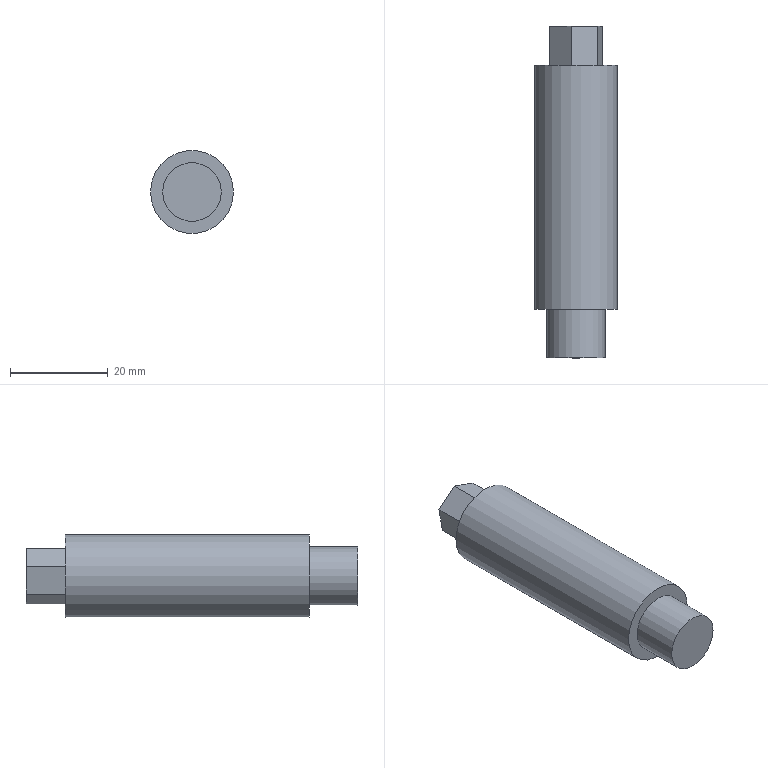Component | NX | STOP_PIN | 1 solid | 12 faces | box 17 x 68 x 17 mm | volume 13173 mm3 | plane 10 | cylinder 2 | commonest cylinder face diameters 12 x1 17 x1
STEP:
#1=CARTESIAN_POINT('',(0.,0.,0.));
#2=DIRECTION('',(0.,0.,1.));
#3=DIRECTION('',(1.,0.,0.));
#4=AXIS2_PLACEMENT_3D('',#1,#2,#3);
#5=CARTESIAN_POINT('',(-15.459,67.5,12.621));
#6=VERTEX_POINT('',#5);
#7=CARTESIAN_POINT('',(-6.959,67.5,12.621));
#8=DIRECTION('',(0.,-1.,0.));
#9=DIRECTION('',(-1.,0.,0.));
#10=AXIS2_PLACEMENT_3D('',#7,#8,#9);
#11=CIRCLE('',#10,8.5);
#12=CARTESIAN_POINT('',(-6.959,67.5,12.621));
#13=DIRECTION('',(0.,-1.,0.));
#14=DIRECTION('',(-1.,0.,0.));
#15=AXIS2_PLACEMENT_3D('',#12,#13,#14);
#16=PLANE('',#15);
#17=CARTESIAN_POINT('',(0.,0.));
#18=DIRECTION('',(1.,0.));
#19=AXIS2_PLACEMENT_2D('',#17,#18);
#20=CIRCLE('',#19,8.5);
#21=(GEOMETRIC_REPRESENTATION_CONTEXT(2)PARAMETRIC_REPRESENTATION_CONTEXT()REPRESENTATION_CONTEXT('',''));
#22=DEFINITIONAL_REPRESENTATION('',(#20),#21);
#23=PCURVE('',#16,#22);
#24=CARTESIAN_POINT('',(-6.959,67.5,12.621));
#25=DIRECTION('',(0.,-1.,0.));
#26=DIRECTION('',(-1.,0.,0.));
#27=AXIS2_PLACEMENT_3D('',#24,#25,#26);
#28=CYLINDRICAL_SURFACE('',#27,8.5);
#29=CARTESIAN_POINT('',(0.,0.));
#30=DIRECTION('',(1.,0.));
#31=VECTOR('',#30,1.);
#32=LINE('',#29,#31);
#33=(GEOMETRIC_REPRESENTATION_CONTEXT(2)PARAMETRIC_REPRESENTATION_CONTEXT()REPRESENTATION_CONTEXT('',''));
#34=DEFINITIONAL_REPRESENTATION('',(#32),#33);
#35=PCURVE('',#28,#34);
#36=SURFACE_CURVE('',#11,(#23,#35),.PCURVE_S1.);
#37=EDGE_CURVE('',#6,#6,#36,.T.);
#38=ORIENTED_EDGE('',*,*,#37,.F.);
#39=EDGE_LOOP('',(#38));
#40=FACE_BOUND('',#39,.T.);
#41=CARTESIAN_POINT('',(-7.962,67.5,18.307));
#42=VERTEX_POINT('',#41);
#43=CARTESIAN_POINT('',(-2.537,67.5,16.333));
#44=VERTEX_POINT('',#43);
#45=CARTESIAN_POINT('',(-7.962,67.5,18.307));
#46=DIRECTION('',(0.9397,0.,-0.342));
#47=VECTOR('',#46,1.);
#48=LINE('',#45,#47);
#49=CARTESIAN_POINT('',(1.003,-5.686));
#50=DIRECTION('',(-0.9397,0.342));
#51=VECTOR('',#50,1.);
#52=LINE('',#49,#51);
#53=(GEOMETRIC_REPRESENTATION_CONTEXT(2)PARAMETRIC_REPRESENTATION_CONTEXT()REPRESENTATION_CONTEXT('',''));
#54=DEFINITIONAL_REPRESENTATION('',(#52),#53);
#55=PCURVE('',#16,#54);
#56=CARTESIAN_POINT('',(-7.962,75.5,18.307));
#57=DIRECTION('',(-0.342,0.,-0.9397));
#58=DIRECTION('',(-0.9397,0.,0.342));
#59=AXIS2_PLACEMENT_3D('',#56,#57,#58);
#60=PLANE('',#59);
#61=CARTESIAN_POINT('',(0.,-8.));
#62=DIRECTION('',(-1.,0.));
#63=VECTOR('',#62,1.);
#64=LINE('',#61,#63);
#65=(GEOMETRIC_REPRESENTATION_CONTEXT(2)PARAMETRIC_REPRESENTATION_CONTEXT()REPRESENTATION_CONTEXT('',''));
#66=DEFINITIONAL_REPRESENTATION('',(#64),#65);
#67=PCURVE('',#60,#66);
#68=SURFACE_CURVE('',#48,(#55,#67),.PCURVE_S1.);
#69=EDGE_CURVE('',#42,#44,#68,.T.);
#70=ORIENTED_EDGE('',*,*,#69,.F.);
#71=CARTESIAN_POINT('',(-12.385,67.5,14.596));
#72=VERTEX_POINT('',#71);
#73=CARTESIAN_POINT('',(-12.385,67.5,14.596));
#74=DIRECTION('',(0.766,0.,0.6428));
#75=VECTOR('',#74,1.);
#76=LINE('',#73,#75);
#77=CARTESIAN_POINT('',(5.425,-1.975));
#78=DIRECTION('',(-0.766,-0.6428));
#79=VECTOR('',#78,1.);
#80=LINE('',#77,#79);
#81=(GEOMETRIC_REPRESENTATION_CONTEXT(2)PARAMETRIC_REPRESENTATION_CONTEXT()REPRESENTATION_CONTEXT('',''));
#82=DEFINITIONAL_REPRESENTATION('',(#80),#81);
#83=PCURVE('',#16,#82);
#84=CARTESIAN_POINT('',(-12.385,75.5,14.596));
#85=DIRECTION('',(0.6428,0.,-0.766));
#86=DIRECTION('',(-0.766,0.,-0.6428));
#87=AXIS2_PLACEMENT_3D('',#84,#85,#86);
#88=PLANE('',#87);
#89=CARTESIAN_POINT('',(0.,-8.));
#90=DIRECTION('',(-1.,0.));
#91=VECTOR('',#90,1.);
#92=LINE('',#89,#91);
#93=(GEOMETRIC_REPRESENTATION_CONTEXT(2)PARAMETRIC_REPRESENTATION_CONTEXT()REPRESENTATION_CONTEXT('',''));
#94=DEFINITIONAL_REPRESENTATION('',(#92),#93);
#95=PCURVE('',#88,#94);
#96=SURFACE_CURVE('',#76,(#83,#95),.PCURVE_S1.);
#97=EDGE_CURVE('',#72,#42,#96,.T.);
#98=ORIENTED_EDGE('',*,*,#97,.F.);
#99=CARTESIAN_POINT('',(-11.382,67.5,8.91));
#100=VERTEX_POINT('',#99);
#101=CARTESIAN_POINT('',(-11.382,67.5,8.91));
#102=DIRECTION('',(-0.1736,0.,0.9848));
#103=VECTOR('',#102,1.);
#104=LINE('',#101,#103);
#105=CARTESIAN_POINT('',(4.423,3.711));
#106=DIRECTION('',(0.1736,-0.9848));
#107=VECTOR('',#106,1.);
#108=LINE('',#105,#107);
#109=(GEOMETRIC_REPRESENTATION_CONTEXT(2)PARAMETRIC_REPRESENTATION_CONTEXT()REPRESENTATION_CONTEXT('',''));
#110=DEFINITIONAL_REPRESENTATION('',(#108),#109);
#111=PCURVE('',#16,#110);
#112=CARTESIAN_POINT('',(-11.382,75.5,8.91));
#113=DIRECTION('',(0.9848,0.,0.1736));
#114=DIRECTION('',(0.1736,0.,-0.9848));
#115=AXIS2_PLACEMENT_3D('',#112,#113,#114);
#116=PLANE('',#115);
#117=CARTESIAN_POINT('',(0.,-8.));
#118=DIRECTION('',(-1.,0.));
#119=VECTOR('',#118,1.);
#120=LINE('',#117,#119);
#121=(GEOMETRIC_REPRESENTATION_CONTEXT(2)PARAMETRIC_REPRESENTATION_CONTEXT()REPRESENTATION_CONTEXT('',''));
#122=DEFINITIONAL_REPRESENTATION('',(#120),#121);
#123=PCURVE('',#116,#122);
#124=SURFACE_CURVE('',#104,(#111,#123),.PCURVE_S1.);
#125=EDGE_CURVE('',#100,#72,#124,.T.);
#126=ORIENTED_EDGE('',*,*,#125,.F.);
#127=CARTESIAN_POINT('',(-5.957,67.5,6.936));
#128=VERTEX_POINT('',#127);
#129=CARTESIAN_POINT('',(-5.957,67.5,6.936));
#130=DIRECTION('',(-0.9397,0.,0.342));
#131=VECTOR('',#130,1.);
#132=LINE('',#129,#131);
#133=CARTESIAN_POINT('',(-1.003,5.686));
#134=DIRECTION('',(0.9397,-0.342));
#135=VECTOR('',#134,1.);
#136=LINE('',#133,#135);
#137=(GEOMETRIC_REPRESENTATION_CONTEXT(2)PARAMETRIC_REPRESENTATION_CONTEXT()REPRESENTATION_CONTEXT('',''));
#138=DEFINITIONAL_REPRESENTATION('',(#136),#137);
#139=PCURVE('',#16,#138);
#140=CARTESIAN_POINT('',(-5.957,75.5,6.936));
#141=DIRECTION('',(0.342,0.,0.9397));
#142=DIRECTION('',(0.9397,0.,-0.342));
#143=AXIS2_PLACEMENT_3D('',#140,#141,#142);
#144=PLANE('',#143);
#145=CARTESIAN_POINT('',(0.,-8.));
#146=DIRECTION('',(-1.,0.));
#147=VECTOR('',#146,1.);
#148=LINE('',#145,#147);
#149=(GEOMETRIC_REPRESENTATION_CONTEXT(2)PARAMETRIC_REPRESENTATION_CONTEXT()REPRESENTATION_CONTEXT('',''));
#150=DEFINITIONAL_REPRESENTATION('',(#148),#149);
#151=PCURVE('',#144,#150);
#152=SURFACE_CURVE('',#132,(#139,#151),.PCURVE_S1.);
#153=EDGE_CURVE('',#128,#100,#152,.T.);
#154=ORIENTED_EDGE('',*,*,#153,.F.);
#155=CARTESIAN_POINT('',(-1.534,67.5,10.647));
#156=VERTEX_POINT('',#155);
#157=CARTESIAN_POINT('',(-1.534,67.5,10.647));
#158=DIRECTION('',(-0.766,0.,-0.6428));
#159=VECTOR('',#158,1.);
#160=LINE('',#157,#159);
#161=CARTESIAN_POINT('',(-5.425,1.975));
#162=DIRECTION('',(0.766,0.6428));
#163=VECTOR('',#162,1.);
#164=LINE('',#161,#163);
#165=(GEOMETRIC_REPRESENTATION_CONTEXT(2)PARAMETRIC_REPRESENTATION_CONTEXT()REPRESENTATION_CONTEXT('',''));
#166=DEFINITIONAL_REPRESENTATION('',(#164),#165);
#167=PCURVE('',#16,#166);
#168=CARTESIAN_POINT('',(-1.534,75.5,10.647));
#169=DIRECTION('',(-0.6428,0.,0.766));
#170=DIRECTION('',(0.766,0.,0.6428));
#171=AXIS2_PLACEMENT_3D('',#168,#169,#170);
#172=PLANE('',#171);
#173=CARTESIAN_POINT('',(0.,-8.));
#174=DIRECTION('',(-1.,0.));
#175=VECTOR('',#174,1.);
#176=LINE('',#173,#175);
#177=(GEOMETRIC_REPRESENTATION_CONTEXT(2)PARAMETRIC_REPRESENTATION_CONTEXT()REPRESENTATION_CONTEXT('',''));
#178=DEFINITIONAL_REPRESENTATION('',(#176),#177);
#179=PCURVE('',#172,#178);
#180=SURFACE_CURVE('',#160,(#167,#179),.PCURVE_S1.);
#181=EDGE_CURVE('',#156,#128,#180,.T.);
#182=ORIENTED_EDGE('',*,*,#181,.F.);
#183=CARTESIAN_POINT('',(-2.537,67.5,16.333));
#184=DIRECTION('',(0.1736,0.,-0.9848));
#185=VECTOR('',#184,1.);
#186=LINE('',#183,#185);
#187=CARTESIAN_POINT('',(-4.423,-3.711));
#188=DIRECTION('',(-0.1736,0.9848));
#189=VECTOR('',#188,1.);
#190=LINE('',#187,#189);
#191=(GEOMETRIC_REPRESENTATION_CONTEXT(2)PARAMETRIC_REPRESENTATION_CONTEXT()REPRESENTATION_CONTEXT('',''));
#192=DEFINITIONAL_REPRESENTATION('',(#190),#191);
#193=PCURVE('',#16,#192);
#194=CARTESIAN_POINT('',(-2.537,75.5,16.333));
#195=DIRECTION('',(-0.9848,0.,-0.1736));
#196=DIRECTION('',(-0.1736,0.,0.9848));
#197=AXIS2_PLACEMENT_3D('',#194,#195,#196);
#198=PLANE('',#197);
#199=CARTESIAN_POINT('',(0.,-8.));
#200=DIRECTION('',(-1.,0.));
#201=VECTOR('',#200,1.);
#202=LINE('',#199,#201);
#203=(GEOMETRIC_REPRESENTATION_CONTEXT(2)PARAMETRIC_REPRESENTATION_CONTEXT()REPRESENTATION_CONTEXT('',''));
#204=DEFINITIONAL_REPRESENTATION('',(#202),#203);
#205=PCURVE('',#198,#204);
#206=SURFACE_CURVE('',#186,(#193,#205),.PCURVE_S1.);
#207=EDGE_CURVE('',#44,#156,#206,.T.);
#208=ORIENTED_EDGE('',*,*,#207,.F.);
#209=EDGE_LOOP('',(#70,#98,#126,#154,#182,#208));
#210=FACE_BOUND('',#209,.T.);
#211=ADVANCED_FACE('',(#40,#210),#16,.F.);
#212=CARTESIAN_POINT('',(-0.9594,17.5,12.621));
#213=VERTEX_POINT('',#212);
#214=CARTESIAN_POINT('',(-6.959,17.5,12.621));
#215=DIRECTION('',(0.,1.,0.));
#216=DIRECTION('',(1.,0.,0.));
#217=AXIS2_PLACEMENT_3D('',#214,#215,#216);
#218=CIRCLE('',#217,6.);
#219=CARTESIAN_POINT('',(-6.959,17.5,12.621));
#220=DIRECTION('',(0.,-1.,0.));
#221=DIRECTION('',(-1.,0.,0.));
#222=AXIS2_PLACEMENT_3D('',#219,#220,#221);
#223=CYLINDRICAL_SURFACE('',#222,6.);
#224=CARTESIAN_POINT('',(9.425,0.));
#225=DIRECTION('',(-1.,0.));
#226=VECTOR('',#225,1.);
#227=LINE('',#224,#226);
#228=(GEOMETRIC_REPRESENTATION_CONTEXT(2)PARAMETRIC_REPRESENTATION_CONTEXT()REPRESENTATION_CONTEXT('',''));
#229=DEFINITIONAL_REPRESENTATION('',(#227),#228);
#230=PCURVE('',#223,#229);
#231=CARTESIAN_POINT('',(-6.959,17.5,12.621));
#232=DIRECTION('',(0.,-1.,0.));
#233=DIRECTION('',(-1.,0.,0.));
#234=AXIS2_PLACEMENT_3D('',#231,#232,#233);
#235=PLANE('',#234);
#236=CARTESIAN_POINT('',(-6.,0.));
#237=CARTESIAN_POINT('',(-6.,10.392));
#238=CARTESIAN_POINT('',(3.,5.196));
#239=CARTESIAN_POINT('',(12.,0.));
#240=CARTESIAN_POINT('',(3.,-5.196));
#241=CARTESIAN_POINT('',(-6.,-10.392));
#242=CARTESIAN_POINT('',(-6.,0.));
#243=(BOUNDED_CURVE()B_SPLINE_CURVE(2,(#236,#237,#238,#239,#240,#241,#242),.UNSPECIFIED.,.T.,.F.)B_SPLINE_CURVE_WITH_KNOTS((1,2,2,2,2,1),(-2.094,0.,2.094,4.189,6.283,8.378),.UNSPECIFIED.)CURVE()GEOMETRIC_REPRESENTATION_ITEM()RATIONAL_B_SPLINE_CURVE((1.,0.5,1.,0.5,1.,0.5,1.))REPRESENTATION_ITEM(''));
#244=(GEOMETRIC_REPRESENTATION_CONTEXT(2)PARAMETRIC_REPRESENTATION_CONTEXT()REPRESENTATION_CONTEXT('',''));
#245=DEFINITIONAL_REPRESENTATION('',(#243),#244);
#246=PCURVE('',#235,#245);
#247=SURFACE_CURVE('',#218,(#230,#246),.PCURVE_S1.);
#248=EDGE_CURVE('',#213,#213,#247,.T.);
#249=ORIENTED_EDGE('',*,*,#248,.F.);
#250=CARTESIAN_POINT('',(-0.9594,7.5,12.621));
#251=VERTEX_POINT('',#250);
#252=CARTESIAN_POINT('',(-0.9594,17.5,12.621));
#253=CARTESIAN_POINT('',(-0.9594,7.5,12.621));
#254=B_SPLINE_CURVE_WITH_KNOTS('',1,(#252,#253),.UNSPECIFIED.,.F.,.F.,(2,2),(0.,10.),.PIECEWISE_BEZIER_KNOTS.);
#255=CARTESIAN_POINT('',(9.425,0.));
#256=DIRECTION('',(0.,1.));
#257=VECTOR('',#256,1.);
#258=LINE('',#255,#257);
#259=(GEOMETRIC_REPRESENTATION_CONTEXT(2)PARAMETRIC_REPRESENTATION_CONTEXT()REPRESENTATION_CONTEXT('',''));
#260=DEFINITIONAL_REPRESENTATION('',(#258),#259);
#261=PCURVE('',#223,#260);
#262=CARTESIAN_POINT('',(3.142,0.));
#263=DIRECTION('',(0.,1.));
#264=VECTOR('',#263,1.);
#265=LINE('',#262,#264);
#266=(GEOMETRIC_REPRESENTATION_CONTEXT(2)PARAMETRIC_REPRESENTATION_CONTEXT()REPRESENTATION_CONTEXT('',''));
#267=DEFINITIONAL_REPRESENTATION('',(#265),#266);
#268=PCURVE('',#223,#267);
#269=SEAM_CURVE('',#254,(#261,#268),.PCURVE_S1.);
#270=EDGE_CURVE('',#213,#251,#269,.T.);
#271=ORIENTED_EDGE('',*,*,#270,.T.);
#272=CARTESIAN_POINT('',(-6.959,7.5,12.621));
#273=DIRECTION('',(0.,1.,0.));
#274=DIRECTION('',(1.,0.,0.));
#275=AXIS2_PLACEMENT_3D('',#272,#273,#274);
#276=CIRCLE('',#275,6.);
#277=CARTESIAN_POINT('',(9.425,10.));
#278=DIRECTION('',(-1.,0.));
#279=VECTOR('',#278,1.);
#280=LINE('',#277,#279);
#281=(GEOMETRIC_REPRESENTATION_CONTEXT(2)PARAMETRIC_REPRESENTATION_CONTEXT()REPRESENTATION_CONTEXT('',''));
#282=DEFINITIONAL_REPRESENTATION('',(#280),#281);
#283=PCURVE('',#223,#282);
#284=CARTESIAN_POINT('',(-6.959,7.5,12.621));
#285=DIRECTION('',(0.,1.,0.));
#286=DIRECTION('',(1.,0.,0.));
#287=AXIS2_PLACEMENT_3D('',#284,#285,#286);
#288=PLANE('',#287);
#289=CARTESIAN_POINT('',(0.,0.));
#290=DIRECTION('',(1.,0.));
#291=AXIS2_PLACEMENT_2D('',#289,#290);
#292=CIRCLE('',#291,6.);
#293=(GEOMETRIC_REPRESENTATION_CONTEXT(2)PARAMETRIC_REPRESENTATION_CONTEXT()REPRESENTATION_CONTEXT('',''));
#294=DEFINITIONAL_REPRESENTATION('',(#292),#293);
#295=PCURVE('',#288,#294);
#296=SURFACE_CURVE('',#276,(#283,#295),.PCURVE_S1.);
#297=EDGE_CURVE('',#251,#251,#296,.T.);
#298=ORIENTED_EDGE('',*,*,#297,.T.);
#299=ORIENTED_EDGE('',*,*,#270,.F.);
#300=EDGE_LOOP('',(#249,#271,#298,#299));
#301=FACE_BOUND('',#300,.T.);
#302=ADVANCED_FACE('',(#301),#223,.T.);
#303=ORIENTED_EDGE('',*,*,#297,.F.);
#304=EDGE_LOOP('',(#303));
#305=FACE_BOUND('',#304,.T.);
#306=ADVANCED_FACE('',(#305),#288,.F.);
#307=ORIENTED_EDGE('',*,*,#37,.T.);
#308=CARTESIAN_POINT('',(-15.459,17.5,12.621));
#309=VERTEX_POINT('',#308);
#310=CARTESIAN_POINT('',(-15.459,67.5,12.621));
#311=CARTESIAN_POINT('',(-15.459,17.5,12.621));
#312=B_SPLINE_CURVE_WITH_KNOTS('',1,(#310,#311),.UNSPECIFIED.,.F.,.F.,(2,2),(0.,50.),.PIECEWISE_BEZIER_KNOTS.);
#313=CARTESIAN_POINT('',(6.283,0.));
#314=DIRECTION('',(0.,1.));
#315=VECTOR('',#314,1.);
#316=LINE('',#313,#315);
#317=(GEOMETRIC_REPRESENTATION_CONTEXT(2)PARAMETRIC_REPRESENTATION_CONTEXT()REPRESENTATION_CONTEXT('',''));
#318=DEFINITIONAL_REPRESENTATION('',(#316),#317);
#319=PCURVE('',#28,#318);
#320=CARTESIAN_POINT('',(0.,0.));
#321=DIRECTION('',(0.,1.));
#322=VECTOR('',#321,1.);
#323=LINE('',#320,#322);
#324=(GEOMETRIC_REPRESENTATION_CONTEXT(2)PARAMETRIC_REPRESENTATION_CONTEXT()REPRESENTATION_CONTEXT('',''));
#325=DEFINITIONAL_REPRESENTATION('',(#323),#324);
#326=PCURVE('',#28,#325);
#327=SEAM_CURVE('',#312,(#319,#326),.PCURVE_S1.);
#328=EDGE_CURVE('',#6,#309,#327,.T.);
#329=ORIENTED_EDGE('',*,*,#328,.T.);
#330=CARTESIAN_POINT('',(-6.959,17.5,12.621));
#331=DIRECTION('',(0.,-1.,0.));
#332=DIRECTION('',(-1.,0.,0.));
#333=AXIS2_PLACEMENT_3D('',#330,#331,#332);
#334=CIRCLE('',#333,8.5);
#335=CARTESIAN_POINT('',(0.,50.));
#336=DIRECTION('',(1.,0.));
#337=VECTOR('',#336,1.);
#338=LINE('',#335,#337);
#339=(GEOMETRIC_REPRESENTATION_CONTEXT(2)PARAMETRIC_REPRESENTATION_CONTEXT()REPRESENTATION_CONTEXT('',''));
#340=DEFINITIONAL_REPRESENTATION('',(#338),#339);
#341=PCURVE('',#28,#340);
#342=CARTESIAN_POINT('',(0.,0.));
#343=DIRECTION('',(1.,0.));
#344=AXIS2_PLACEMENT_2D('',#342,#343);
#345=CIRCLE('',#344,8.5);
#346=(GEOMETRIC_REPRESENTATION_CONTEXT(2)PARAMETRIC_REPRESENTATION_CONTEXT()REPRESENTATION_CONTEXT('',''));
#347=DEFINITIONAL_REPRESENTATION('',(#345),#346);
#348=PCURVE('',#235,#347);
#349=SURFACE_CURVE('',#334,(#341,#348),.PCURVE_S1.);
#350=EDGE_CURVE('',#309,#309,#349,.T.);
#351=ORIENTED_EDGE('',*,*,#350,.F.);
#352=ORIENTED_EDGE('',*,*,#328,.F.);
#353=EDGE_LOOP('',(#307,#329,#351,#352));
#354=FACE_BOUND('',#353,.T.);
#355=ADVANCED_FACE('',(#354),#28,.T.);
#356=ORIENTED_EDGE('',*,*,#248,.T.);
#357=EDGE_LOOP('',(#356));
#358=FACE_BOUND('',#357,.T.);
#359=ORIENTED_EDGE('',*,*,#350,.T.);
#360=EDGE_LOOP('',(#359));
#361=FACE_BOUND('',#360,.T.);
#362=ADVANCED_FACE('',(#358,#361),#235,.T.);
#363=ORIENTED_EDGE('',*,*,#69,.T.);
#364=CARTESIAN_POINT('',(-2.537,75.5,16.333));
#365=VERTEX_POINT('',#364);
#366=CARTESIAN_POINT('',(-2.537,75.5,16.333));
#367=DIRECTION('',(0.,-1.,0.));
#368=VECTOR('',#367,1.);
#369=LINE('',#366,#368);
#370=CARTESIAN_POINT('',(-5.774,0.));
#371=DIRECTION('',(0.,-1.));
#372=VECTOR('',#371,1.);
#373=LINE('',#370,#372);
#374=(GEOMETRIC_REPRESENTATION_CONTEXT(2)PARAMETRIC_REPRESENTATION_CONTEXT()REPRESENTATION_CONTEXT('',''));
#375=DEFINITIONAL_REPRESENTATION('',(#373),#374);
#376=PCURVE('',#60,#375);
#377=CARTESIAN_POINT('',(0.,0.));
#378=DIRECTION('',(0.,-1.));
#379=VECTOR('',#378,1.);
#380=LINE('',#377,#379);
#381=(GEOMETRIC_REPRESENTATION_CONTEXT(2)PARAMETRIC_REPRESENTATION_CONTEXT()REPRESENTATION_CONTEXT('',''));
#382=DEFINITIONAL_REPRESENTATION('',(#380),#381);
#383=PCURVE('',#198,#382);
#384=SURFACE_CURVE('',#369,(#376,#383),.PCURVE_S1.);
#385=EDGE_CURVE('',#365,#44,#384,.T.);
#386=ORIENTED_EDGE('',*,*,#385,.F.);
#387=CARTESIAN_POINT('',(-7.962,75.5,18.307));
#388=VERTEX_POINT('',#387);
#389=CARTESIAN_POINT('',(-7.962,75.5,18.307));
#390=DIRECTION('',(0.9397,0.,-0.342));
#391=VECTOR('',#390,1.);
#392=LINE('',#389,#391);
#393=CARTESIAN_POINT('',(0.,0.));
#394=DIRECTION('',(-1.,0.));
#395=VECTOR('',#394,1.);
#396=LINE('',#393,#395);
#397=(GEOMETRIC_REPRESENTATION_CONTEXT(2)PARAMETRIC_REPRESENTATION_CONTEXT()REPRESENTATION_CONTEXT('',''));
#398=DEFINITIONAL_REPRESENTATION('',(#396),#397);
#399=PCURVE('',#60,#398);
#400=CARTESIAN_POINT('',(-6.959,75.5,12.621));
#401=DIRECTION('',(0.,1.,0.));
#402=DIRECTION('',(1.,0.,0.));
#403=AXIS2_PLACEMENT_3D('',#400,#401,#402);
#404=PLANE('',#403);
#405=CARTESIAN_POINT('',(-1.003,-5.686));
#406=DIRECTION('',(0.9397,0.342));
#407=VECTOR('',#406,1.);
#408=LINE('',#405,#407);
#409=(GEOMETRIC_REPRESENTATION_CONTEXT(2)PARAMETRIC_REPRESENTATION_CONTEXT()REPRESENTATION_CONTEXT('',''));
#410=DEFINITIONAL_REPRESENTATION('',(#408),#409);
#411=PCURVE('',#404,#410);
#412=SURFACE_CURVE('',#392,(#399,#411),.PCURVE_S1.);
#413=EDGE_CURVE('',#388,#365,#412,.T.);
#414=ORIENTED_EDGE('',*,*,#413,.F.);
#415=CARTESIAN_POINT('',(-7.962,75.5,18.307));
#416=DIRECTION('',(0.,-1.,0.));
#417=VECTOR('',#416,1.);
#418=LINE('',#415,#417);
#419=CARTESIAN_POINT('',(0.,0.));
#420=DIRECTION('',(0.,-1.));
#421=VECTOR('',#420,1.);
#422=LINE('',#419,#421);
#423=(GEOMETRIC_REPRESENTATION_CONTEXT(2)PARAMETRIC_REPRESENTATION_CONTEXT()REPRESENTATION_CONTEXT('',''));
#424=DEFINITIONAL_REPRESENTATION('',(#422),#423);
#425=PCURVE('',#60,#424);
#426=CARTESIAN_POINT('',(-5.774,0.));
#427=DIRECTION('',(0.,-1.));
#428=VECTOR('',#427,1.);
#429=LINE('',#426,#428);
#430=(GEOMETRIC_REPRESENTATION_CONTEXT(2)PARAMETRIC_REPRESENTATION_CONTEXT()REPRESENTATION_CONTEXT('',''));
#431=DEFINITIONAL_REPRESENTATION('',(#429),#430);
#432=PCURVE('',#88,#431);
#433=SURFACE_CURVE('',#418,(#425,#432),.PCURVE_S1.);
#434=EDGE_CURVE('',#388,#42,#433,.T.);
#435=ORIENTED_EDGE('',*,*,#434,.T.);
#436=EDGE_LOOP('',(#363,#386,#414,#435));
#437=FACE_BOUND('',#436,.T.);
#438=ADVANCED_FACE('',(#437),#60,.F.);
#439=ORIENTED_EDGE('',*,*,#207,.T.);
#440=CARTESIAN_POINT('',(-1.534,75.5,10.647));
#441=VERTEX_POINT('',#440);
#442=CARTESIAN_POINT('',(-1.534,75.5,10.647));
#443=DIRECTION('',(0.,-1.,0.));
#444=VECTOR('',#443,1.);
#445=LINE('',#442,#444);
#446=CARTESIAN_POINT('',(-5.774,0.));
#447=DIRECTION('',(0.,-1.));
#448=VECTOR('',#447,1.);
#449=LINE('',#446,#448);
#450=(GEOMETRIC_REPRESENTATION_CONTEXT(2)PARAMETRIC_REPRESENTATION_CONTEXT()REPRESENTATION_CONTEXT('',''));
#451=DEFINITIONAL_REPRESENTATION('',(#449),#450);
#452=PCURVE('',#198,#451);
#453=CARTESIAN_POINT('',(0.,0.));
#454=DIRECTION('',(0.,-1.));
#455=VECTOR('',#454,1.);
#456=LINE('',#453,#455);
#457=(GEOMETRIC_REPRESENTATION_CONTEXT(2)PARAMETRIC_REPRESENTATION_CONTEXT()REPRESENTATION_CONTEXT('',''));
#458=DEFINITIONAL_REPRESENTATION('',(#456),#457);
#459=PCURVE('',#172,#458);
#460=SURFACE_CURVE('',#445,(#452,#459),.PCURVE_S1.);
#461=EDGE_CURVE('',#441,#156,#460,.T.);
#462=ORIENTED_EDGE('',*,*,#461,.F.);
#463=CARTESIAN_POINT('',(-2.537,75.5,16.333));
#464=DIRECTION('',(0.1736,0.,-0.9848));
#465=VECTOR('',#464,1.);
#466=LINE('',#463,#465);
#467=CARTESIAN_POINT('',(0.,0.));
#468=DIRECTION('',(-1.,0.));
#469=VECTOR('',#468,1.);
#470=LINE('',#467,#469);
#471=(GEOMETRIC_REPRESENTATION_CONTEXT(2)PARAMETRIC_REPRESENTATION_CONTEXT()REPRESENTATION_CONTEXT('',''));
#472=DEFINITIONAL_REPRESENTATION('',(#470),#471);
#473=PCURVE('',#198,#472);
#474=CARTESIAN_POINT('',(4.423,-3.711));
#475=DIRECTION('',(0.1736,0.9848));
#476=VECTOR('',#475,1.);
#477=LINE('',#474,#476);
#478=(GEOMETRIC_REPRESENTATION_CONTEXT(2)PARAMETRIC_REPRESENTATION_CONTEXT()REPRESENTATION_CONTEXT('',''));
#479=DEFINITIONAL_REPRESENTATION('',(#477),#478);
#480=PCURVE('',#404,#479);
#481=SURFACE_CURVE('',#466,(#473,#480),.PCURVE_S1.);
#482=EDGE_CURVE('',#365,#441,#481,.T.);
#483=ORIENTED_EDGE('',*,*,#482,.F.);
#484=ORIENTED_EDGE('',*,*,#385,.T.);
#485=EDGE_LOOP('',(#439,#462,#483,#484));
#486=FACE_BOUND('',#485,.T.);
#487=ADVANCED_FACE('',(#486),#198,.F.);
#488=ORIENTED_EDGE('',*,*,#181,.T.);
#489=CARTESIAN_POINT('',(-5.957,75.5,6.936));
#490=VERTEX_POINT('',#489);
#491=CARTESIAN_POINT('',(-5.957,75.5,6.936));
#492=DIRECTION('',(0.,-1.,0.));
#493=VECTOR('',#492,1.);
#494=LINE('',#491,#493);
#495=CARTESIAN_POINT('',(-5.774,0.));
#496=DIRECTION('',(0.,-1.));
#497=VECTOR('',#496,1.);
#498=LINE('',#495,#497);
#499=(GEOMETRIC_REPRESENTATION_CONTEXT(2)PARAMETRIC_REPRESENTATION_CONTEXT()REPRESENTATION_CONTEXT('',''));
#500=DEFINITIONAL_REPRESENTATION('',(#498),#499);
#501=PCURVE('',#172,#500);
#502=CARTESIAN_POINT('',(0.,0.));
#503=DIRECTION('',(0.,-1.));
#504=VECTOR('',#503,1.);
#505=LINE('',#502,#504);
#506=(GEOMETRIC_REPRESENTATION_CONTEXT(2)PARAMETRIC_REPRESENTATION_CONTEXT()REPRESENTATION_CONTEXT('',''));
#507=DEFINITIONAL_REPRESENTATION('',(#505),#506);
#508=PCURVE('',#144,#507);
#509=SURFACE_CURVE('',#494,(#501,#508),.PCURVE_S1.);
#510=EDGE_CURVE('',#490,#128,#509,.T.);
#511=ORIENTED_EDGE('',*,*,#510,.F.);
#512=CARTESIAN_POINT('',(-1.534,75.5,10.647));
#513=DIRECTION('',(-0.766,0.,-0.6428));
#514=VECTOR('',#513,1.);
#515=LINE('',#512,#514);
#516=CARTESIAN_POINT('',(0.,0.));
#517=DIRECTION('',(-1.,0.));
#518=VECTOR('',#517,1.);
#519=LINE('',#516,#518);
#520=(GEOMETRIC_REPRESENTATION_CONTEXT(2)PARAMETRIC_REPRESENTATION_CONTEXT()REPRESENTATION_CONTEXT('',''));
#521=DEFINITIONAL_REPRESENTATION('',(#519),#520);
#522=PCURVE('',#172,#521);
#523=CARTESIAN_POINT('',(5.425,1.975));
#524=DIRECTION('',(-0.766,0.6428));
#525=VECTOR('',#524,1.);
#526=LINE('',#523,#525);
#527=(GEOMETRIC_REPRESENTATION_CONTEXT(2)PARAMETRIC_REPRESENTATION_CONTEXT()REPRESENTATION_CONTEXT('',''));
#528=DEFINITIONAL_REPRESENTATION('',(#526),#527);
#529=PCURVE('',#404,#528);
#530=SURFACE_CURVE('',#515,(#522,#529),.PCURVE_S1.);
#531=EDGE_CURVE('',#441,#490,#530,.T.);
#532=ORIENTED_EDGE('',*,*,#531,.F.);
#533=ORIENTED_EDGE('',*,*,#461,.T.);
#534=EDGE_LOOP('',(#488,#511,#532,#533));
#535=FACE_BOUND('',#534,.T.);
#536=ADVANCED_FACE('',(#535),#172,.F.);
#537=ORIENTED_EDGE('',*,*,#153,.T.);
#538=CARTESIAN_POINT('',(-11.382,75.5,8.91));
#539=VERTEX_POINT('',#538);
#540=CARTESIAN_POINT('',(-11.382,75.5,8.91));
#541=DIRECTION('',(0.,-1.,0.));
#542=VECTOR('',#541,1.);
#543=LINE('',#540,#542);
#544=CARTESIAN_POINT('',(-5.774,0.));
#545=DIRECTION('',(0.,-1.));
#546=VECTOR('',#545,1.);
#547=LINE('',#544,#546);
#548=(GEOMETRIC_REPRESENTATION_CONTEXT(2)PARAMETRIC_REPRESENTATION_CONTEXT()REPRESENTATION_CONTEXT('',''));
#549=DEFINITIONAL_REPRESENTATION('',(#547),#548);
#550=PCURVE('',#144,#549);
#551=CARTESIAN_POINT('',(-0.,0.));
#552=DIRECTION('',(0.,-1.));
#553=VECTOR('',#552,1.);
#554=LINE('',#551,#553);
#555=(GEOMETRIC_REPRESENTATION_CONTEXT(2)PARAMETRIC_REPRESENTATION_CONTEXT()REPRESENTATION_CONTEXT('',''));
#556=DEFINITIONAL_REPRESENTATION('',(#554),#555);
#557=PCURVE('',#116,#556);
#558=SURFACE_CURVE('',#543,(#550,#557),.PCURVE_S1.);
#559=EDGE_CURVE('',#539,#100,#558,.T.);
#560=ORIENTED_EDGE('',*,*,#559,.F.);
#561=CARTESIAN_POINT('',(-5.957,75.5,6.936));
#562=DIRECTION('',(-0.9397,0.,0.342));
#563=VECTOR('',#562,1.);
#564=LINE('',#561,#563);
#565=CARTESIAN_POINT('',(0.,0.));
#566=DIRECTION('',(-1.,0.));
#567=VECTOR('',#566,1.);
#568=LINE('',#565,#567);
#569=(GEOMETRIC_REPRESENTATION_CONTEXT(2)PARAMETRIC_REPRESENTATION_CONTEXT()REPRESENTATION_CONTEXT('',''));
#570=DEFINITIONAL_REPRESENTATION('',(#568),#569);
#571=PCURVE('',#144,#570);
#572=CARTESIAN_POINT('',(1.003,5.686));
#573=DIRECTION('',(-0.9397,-0.342));
#574=VECTOR('',#573,1.);
#575=LINE('',#572,#574);
#576=(GEOMETRIC_REPRESENTATION_CONTEXT(2)PARAMETRIC_REPRESENTATION_CONTEXT()REPRESENTATION_CONTEXT('',''));
#577=DEFINITIONAL_REPRESENTATION('',(#575),#576);
#578=PCURVE('',#404,#577);
#579=SURFACE_CURVE('',#564,(#571,#578),.PCURVE_S1.);
#580=EDGE_CURVE('',#490,#539,#579,.T.);
#581=ORIENTED_EDGE('',*,*,#580,.F.);
#582=ORIENTED_EDGE('',*,*,#510,.T.);
#583=EDGE_LOOP('',(#537,#560,#581,#582));
#584=FACE_BOUND('',#583,.T.);
#585=ADVANCED_FACE('',(#584),#144,.F.);
#586=ORIENTED_EDGE('',*,*,#125,.T.);
#587=CARTESIAN_POINT('',(-12.385,75.5,14.596));
#588=VERTEX_POINT('',#587);
#589=CARTESIAN_POINT('',(-12.385,75.5,14.596));
#590=DIRECTION('',(0.,-1.,0.));
#591=VECTOR('',#590,1.);
#592=LINE('',#589,#591);
#593=CARTESIAN_POINT('',(-5.774,0.));
#594=DIRECTION('',(0.,-1.));
#595=VECTOR('',#594,1.);
#596=LINE('',#593,#595);
#597=(GEOMETRIC_REPRESENTATION_CONTEXT(2)PARAMETRIC_REPRESENTATION_CONTEXT()REPRESENTATION_CONTEXT('',''));
#598=DEFINITIONAL_REPRESENTATION('',(#596),#597);
#599=PCURVE('',#116,#598);
#600=CARTESIAN_POINT('',(0.,0.));
#601=DIRECTION('',(0.,-1.));
#602=VECTOR('',#601,1.);
#603=LINE('',#600,#602);
#604=(GEOMETRIC_REPRESENTATION_CONTEXT(2)PARAMETRIC_REPRESENTATION_CONTEXT()REPRESENTATION_CONTEXT('',''));
#605=DEFINITIONAL_REPRESENTATION('',(#603),#604);
#606=PCURVE('',#88,#605);
#607=SURFACE_CURVE('',#592,(#599,#606),.PCURVE_S1.);
#608=EDGE_CURVE('',#588,#72,#607,.T.);
#609=ORIENTED_EDGE('',*,*,#608,.F.);
#610=CARTESIAN_POINT('',(-11.382,75.5,8.91));
#611=DIRECTION('',(-0.1736,0.,0.9848));
#612=VECTOR('',#611,1.);
#613=LINE('',#610,#612);
#614=CARTESIAN_POINT('',(0.,0.));
#615=DIRECTION('',(-1.,0.));
#616=VECTOR('',#615,1.);
#617=LINE('',#614,#616);
#618=(GEOMETRIC_REPRESENTATION_CONTEXT(2)PARAMETRIC_REPRESENTATION_CONTEXT()REPRESENTATION_CONTEXT('',''));
#619=DEFINITIONAL_REPRESENTATION('',(#617),#618);
#620=PCURVE('',#116,#619);
#621=CARTESIAN_POINT('',(-4.423,3.711));
#622=DIRECTION('',(-0.1736,-0.9848));
#623=VECTOR('',#622,1.);
#624=LINE('',#621,#623);
#625=(GEOMETRIC_REPRESENTATION_CONTEXT(2)PARAMETRIC_REPRESENTATION_CONTEXT()REPRESENTATION_CONTEXT('',''));
#626=DEFINITIONAL_REPRESENTATION('',(#624),#625);
#627=PCURVE('',#404,#626);
#628=SURFACE_CURVE('',#613,(#620,#627),.PCURVE_S1.);
#629=EDGE_CURVE('',#539,#588,#628,.T.);
#630=ORIENTED_EDGE('',*,*,#629,.F.);
#631=ORIENTED_EDGE('',*,*,#559,.T.);
#632=EDGE_LOOP('',(#586,#609,#630,#631));
#633=FACE_BOUND('',#632,.T.);
#634=ADVANCED_FACE('',(#633),#116,.F.);
#635=ORIENTED_EDGE('',*,*,#97,.T.);
#636=ORIENTED_EDGE('',*,*,#434,.F.);
#637=CARTESIAN_POINT('',(-12.385,75.5,14.596));
#638=DIRECTION('',(0.766,0.,0.6428));
#639=VECTOR('',#638,1.);
#640=LINE('',#637,#639);
#641=CARTESIAN_POINT('',(0.,0.));
#642=DIRECTION('',(-1.,0.));
#643=VECTOR('',#642,1.);
#644=LINE('',#641,#643);
#645=(GEOMETRIC_REPRESENTATION_CONTEXT(2)PARAMETRIC_REPRESENTATION_CONTEXT()REPRESENTATION_CONTEXT('',''));
#646=DEFINITIONAL_REPRESENTATION('',(#644),#645);
#647=PCURVE('',#88,#646);
#648=CARTESIAN_POINT('',(-5.425,-1.975));
#649=DIRECTION('',(0.766,-0.6428));
#650=VECTOR('',#649,1.);
#651=LINE('',#648,#650);
#652=(GEOMETRIC_REPRESENTATION_CONTEXT(2)PARAMETRIC_REPRESENTATION_CONTEXT()REPRESENTATION_CONTEXT('',''));
#653=DEFINITIONAL_REPRESENTATION('',(#651),#652);
#654=PCURVE('',#404,#653);
#655=SURFACE_CURVE('',#640,(#647,#654),.PCURVE_S1.);
#656=EDGE_CURVE('',#588,#388,#655,.T.);
#657=ORIENTED_EDGE('',*,*,#656,.F.);
#658=ORIENTED_EDGE('',*,*,#608,.T.);
#659=EDGE_LOOP('',(#635,#636,#657,#658));
#660=FACE_BOUND('',#659,.T.);
#661=ADVANCED_FACE('',(#660),#88,.F.);
#662=ORIENTED_EDGE('',*,*,#413,.T.);
#663=ORIENTED_EDGE('',*,*,#482,.T.);
#664=ORIENTED_EDGE('',*,*,#531,.T.);
#665=ORIENTED_EDGE('',*,*,#580,.T.);
#666=ORIENTED_EDGE('',*,*,#629,.T.);
#667=ORIENTED_EDGE('',*,*,#656,.T.);
#668=EDGE_LOOP('',(#662,#663,#664,#665,#666,#667));
#669=FACE_BOUND('',#668,.T.);
#670=ADVANCED_FACE('',(#669),#404,.T.);
#671=CLOSED_SHELL('',(#211,#302,#306,#355,#362,#438,#487,#536,#585,#634,#661,#670));
#672=MANIFOLD_SOLID_BREP('',#671);
#673=(LENGTH_UNIT()NAMED_UNIT(*)SI_UNIT(.MILLI.,.METRE.));
#674=UNCERTAINTY_MEASURE_WITH_UNIT(LENGTH_MEASURE(0.000002),#673,'','');
#675=(NAMED_UNIT(*)PLANE_ANGLE_UNIT()SI_UNIT($,.RADIAN.));
#676=(NAMED_UNIT(*)SI_UNIT($,.STERADIAN.)SOLID_ANGLE_UNIT());
#677=(GEOMETRIC_REPRESENTATION_CONTEXT(3)GLOBAL_UNCERTAINTY_ASSIGNED_CONTEXT((#674))GLOBAL_UNIT_ASSIGNED_CONTEXT((#673,#675,#676))REPRESENTATION_CONTEXT('',''));
#678=ADVANCED_BREP_SHAPE_REPRESENTATION('',(#4,#672),#677);